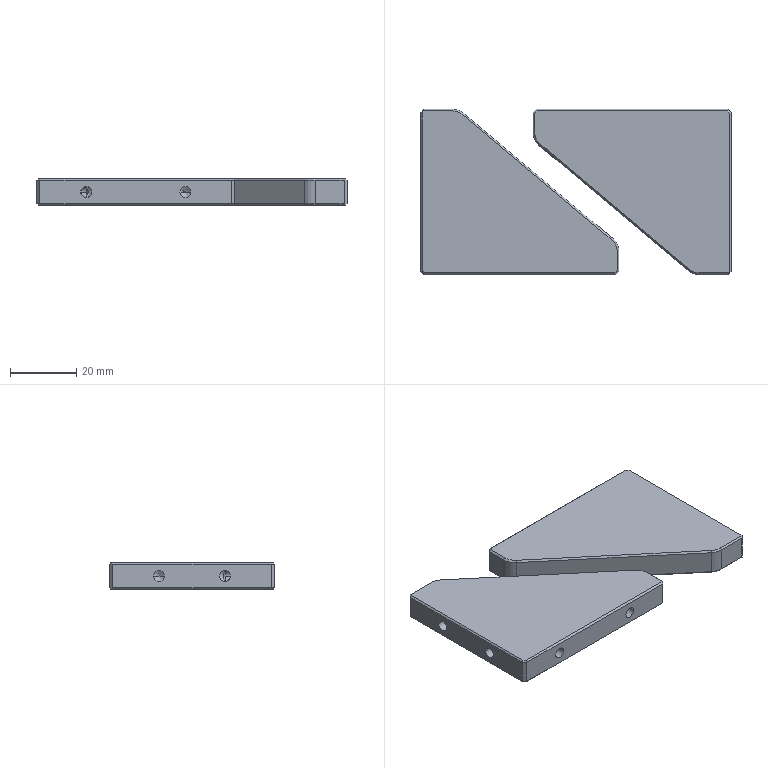CAM job | Mastercam | mm | 8 operations | part box 94 x 50 x 8
1. Contour (Ramp) | 6 - 6 平底刀
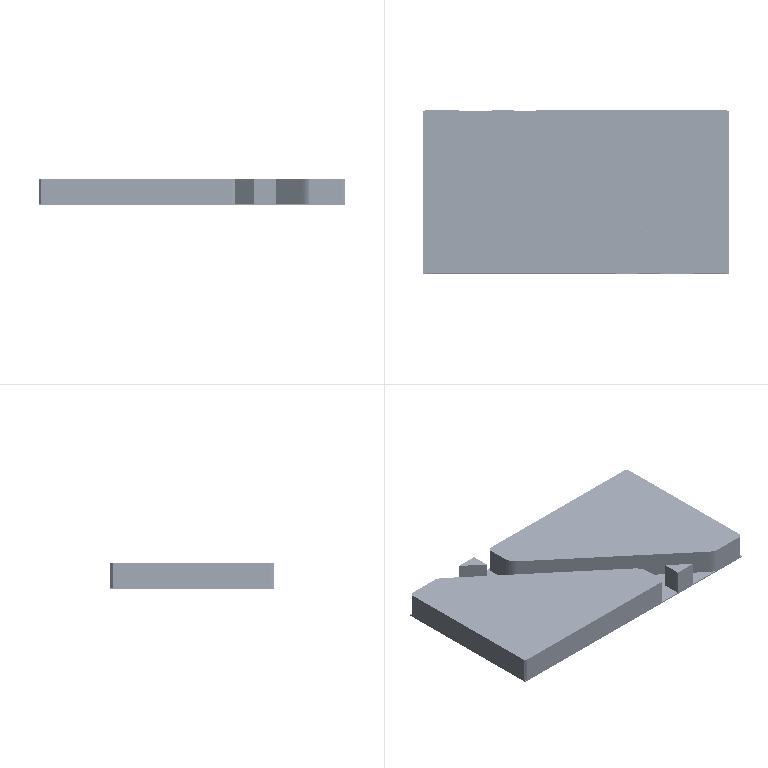2. Contour (2D) | 7 - 4 平底刀
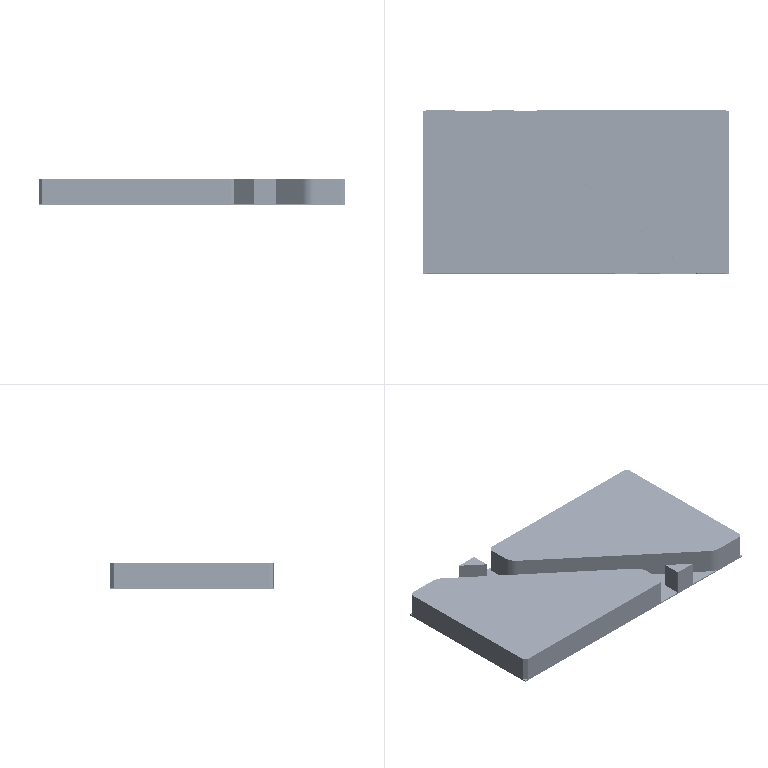3. Contour (2D chamfer) | 2 - 6定位倒角
4. Contour (2D) | 7 - 4 平底刀
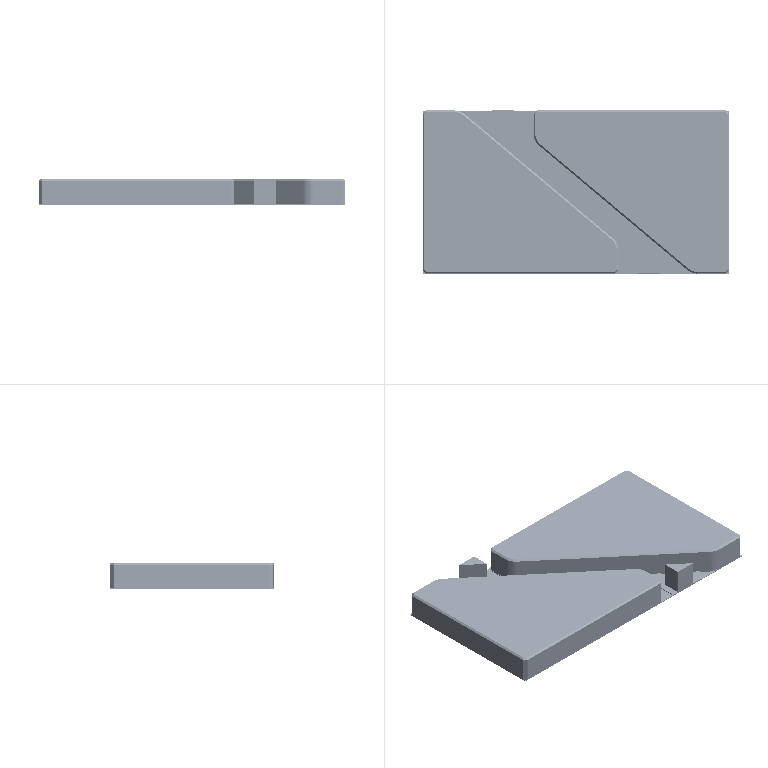5. Drill/Counterbore | 2 - 6定位倒角
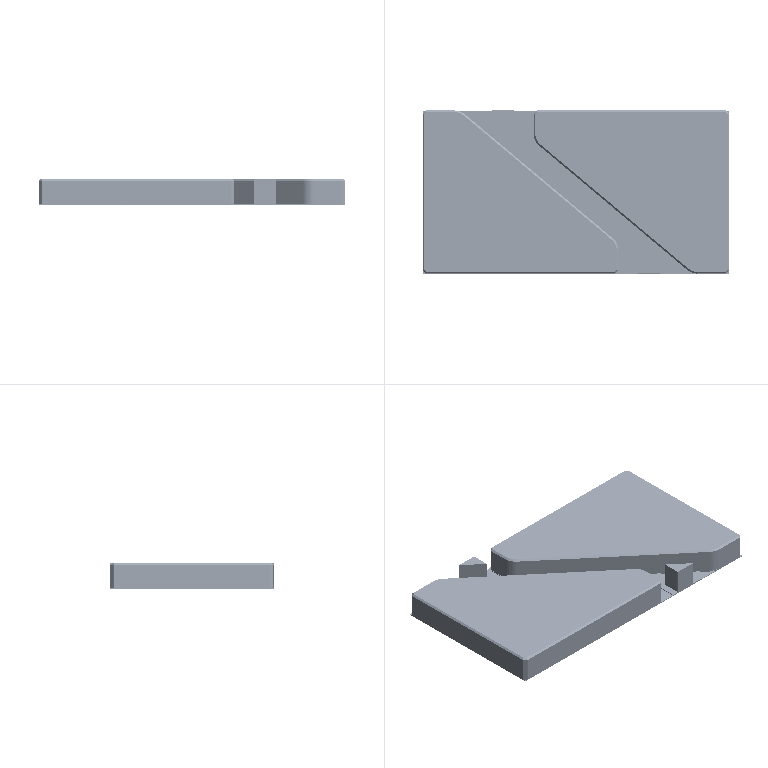6. Peck Drill | 12 - 3.3 钻头
7. Drill/Counterbore | 2 - 6定位倒角
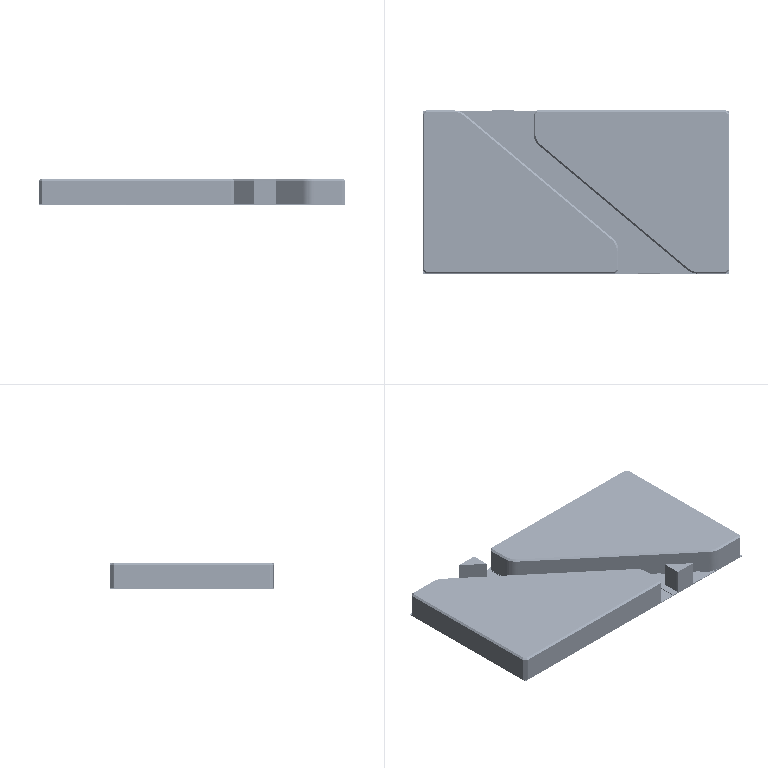8. Peck Drill | 12 - 3.3 钻头